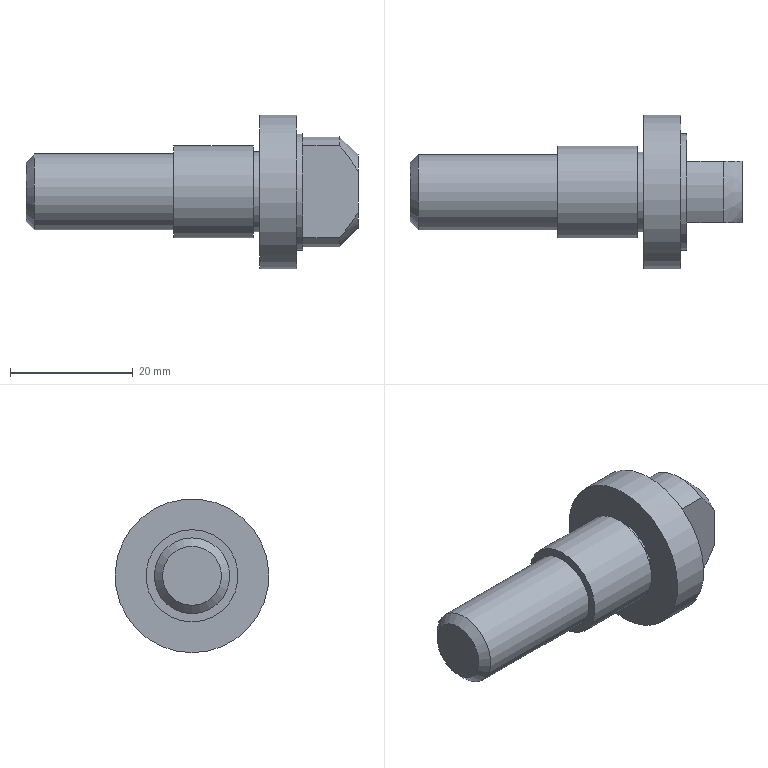Component | NX | REPL_LOC_PIN | 1 solid | 19 faces | volume 9912 mm3 | plane 9 | cylinder 7 | cone 3 | commonest cylinder face diameters 18 x2 12.3 x1 15 x1 13 x1 25 x1 19 x1